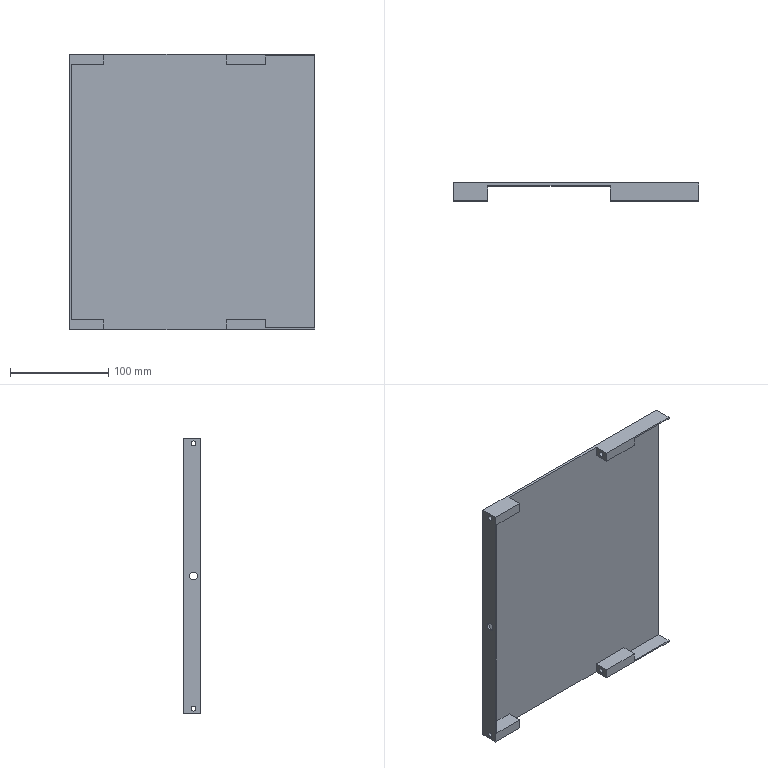Component | SolidWorks | SlideTablePlatform-1 | 1 solid | 32 faces | box 250 x 18 x 280 mm | volume 239541 mm3 | plane 22 | cylinder 10 | commonest cylinder face diameters 5 x8 8 x2
build123d program:
from build123d import *

# Parameters (mm, degrees)
SKETCH1_W           = 250
SKETCH1_H           = 280
BOSS_EXTRUDE1_DEPTH = 1.5
SKETCH2_W           = 35
SKETCH2_H           = 10
SKETCH2_W_2         = 40
BOSS_EXTRUDE2_DEPTH = 15
SKETCH3_R           = 2.5
CUT_EXTRUDE1_DEPTH  = 245.688
SKETCH4_W           = 50
SKETCH4_H           = 1.5
SKETCH4_W_2         = 2
SKETCH4_H_2         = 260
SKETCH4_H_3         = 1.549
BOSS_EXTRUDE3_DEPTH = 15
SKETCH5_R           = 4
CUT_EXTRUDE2_DEPTH  = 10


with BuildPart() as part:
    # Sketch1 → Boss-Extrude1 (new, symmetric)
    with BuildSketch(Plane(origin=(0, 0, 0), x_dir=(1, 0, 0), z_dir=(0, 1, 0))):
        Rectangle(SKETCH1_W, SKETCH1_H)
    extrude(amount=BOSS_EXTRUDE1_DEPTH, both=True)

    # Sketch2 → Boss-Extrude2 (add)
    with BuildSketch(Plane.XZ.offset(1.5)):
        with Locations((107.5, 135)):
            Rectangle(SKETCH2_W, SKETCH2_H)
        with Locations((107.5, -135)):
            Rectangle(SKETCH2_W, SKETCH2_H)
        with Locations((-55, 135)):
            Rectangle(SKETCH2_W_2, SKETCH2_H)
        with Locations((-55, -135)):
            Rectangle(SKETCH2_W_2, SKETCH2_H)
    extrude(amount=BOSS_EXTRUDE2_DEPTH)

    # Sketch3 → Cut-Extrude1 (cut, through all)
    with BuildSketch(Plane.ZY.offset(75)):
        with Locations((-135, -9)):
            Circle(SKETCH3_R)
        with Locations((135, -9)):
            Circle(SKETCH3_R)
    extrude(amount=-CUT_EXTRUDE1_DEPTH, mode=Mode.SUBTRACT)

    # Sketch4 → Boss-Extrude3 (add)
    with BuildSketch(Plane.XZ.offset(1.5)):
        with Locations((-100, -139.25)):
            Rectangle(SKETCH4_W, SKETCH4_H)
        with Locations((124, 0)):
            Rectangle(SKETCH4_W_2, SKETCH4_H_2)
        with Locations((-100, 139.225)):
            Rectangle(SKETCH4_W, SKETCH4_H_3)
    extrude(amount=BOSS_EXTRUDE3_DEPTH)

    # Sketch5 → Cut-Extrude2 (cut)
    with BuildSketch(Plane(origin=(125, 0, 0), x_dir=(0, 0, -1), z_dir=(1, 0, 0))):
        with Locations((0, -9)):
            Circle(SKETCH5_R)
    extrude(amount=-CUT_EXTRUDE2_DEPTH, mode=Mode.SUBTRACT)


solid = part.part

# Placed as in the assembly
solid = solid.moved(Location((157.663, 229, -10), (-180, 0, 180)))
STEP:
#1=COLOUR_RGB('',0.7922,0.8196,0.9333);
#2=FILL_AREA_STYLE_COLOUR('',#1);
#3=FILL_AREA_STYLE('',(#2));
#4=SURFACE_STYLE_FILL_AREA(#3);
#5=SURFACE_SIDE_STYLE('',(#4));
#6=SURFACE_STYLE_USAGE(.BOTH.,#5);
#7=PRESENTATION_STYLE_ASSIGNMENT((#6));
#8=CARTESIAN_POINT('',(1.365,8.661,-0.5512));
#9=VERTEX_POINT('',#8);
#10=CARTESIAN_POINT('',(1.365,8.661,-0.2362));
#11=VERTEX_POINT('',#10);
#12=CARTESIAN_POINT('',(1.365,8.661,-0.3937));
#13=DIRECTION('',(-1.,-0.,-0.));
#14=DIRECTION('',(-0.,0.,1.));
#15=AXIS2_PLACEMENT_3D('',#12,#13,#14);
#16=CIRCLE('',#15,0.1575);
#17=EDGE_CURVE('',#9,#11,#16,.T.);
#18=ORIENTED_EDGE('',*,*,#17,.F.);
#19=CARTESIAN_POINT('',(1.286,8.661,-0.5512));
#20=VERTEX_POINT('',#19);
#21=CARTESIAN_POINT('',(1.68,8.661,-0.5512));
#22=DIRECTION('',(-1.,-0.,-0.));
#23=VECTOR('',#22,39.37);
#24=LINE('',#21,#23);
#25=EDGE_CURVE('',#9,#20,#24,.T.);
#26=ORIENTED_EDGE('',*,*,#25,.T.);
#27=CARTESIAN_POINT('',(1.286,8.661,-0.2362));
#28=VERTEX_POINT('',#27);
#29=CARTESIAN_POINT('',(1.286,8.661,-0.3937));
#30=DIRECTION('',(-1.,-0.,-0.));
#31=DIRECTION('',(-0.,0.,1.));
#32=AXIS2_PLACEMENT_3D('',#29,#30,#31);
#33=CIRCLE('',#32,0.1575);
#34=EDGE_CURVE('',#20,#28,#33,.T.);
#35=ORIENTED_EDGE('',*,*,#34,.T.);
#36=CARTESIAN_POINT('',(1.68,8.661,-0.2362));
#37=DIRECTION('',(-1.,-0.,-0.));
#38=VECTOR('',#37,39.37);
#39=LINE('',#36,#38);
#40=EDGE_CURVE('',#11,#28,#39,.T.);
#41=ORIENTED_EDGE('',*,*,#40,.F.);
#42=EDGE_LOOP('',(#18,#26,#35,#41));
#43=FACE_OUTER_BOUND('',#42,.T.);
#44=CARTESIAN_POINT('',(1.68,8.661,-0.3937));
#45=DIRECTION('',(-1.,-0.,-0.));
#46=DIRECTION('',(-0.,0.,1.));
#47=AXIS2_PLACEMENT_3D('',#44,#45,#46);
#48=CYLINDRICAL_SURFACE('',#47,0.1575);
#49=ADVANCED_FACE('',(#43),#48,.F.);
#50=CARTESIAN_POINT('',(1.286,8.661,-5.61));
#51=VERTEX_POINT('',#50);
#52=CARTESIAN_POINT('',(1.286,8.661,-5.807));
#53=VERTEX_POINT('',#52);
#54=CARTESIAN_POINT('',(1.286,8.661,-5.709));
#55=DIRECTION('',(1.,0.,-0.));
#56=DIRECTION('',(0.,0.,-1.));
#57=AXIS2_PLACEMENT_3D('',#54,#55,#56);
#58=CIRCLE('',#57,0.09843);
#59=EDGE_CURVE('',#51,#53,#58,.T.);
#60=ORIENTED_EDGE('',*,*,#59,.F.);
#61=CARTESIAN_POINT('',(2.664,8.661,-5.61));
#62=VERTEX_POINT('',#61);
#63=CARTESIAN_POINT('',(1.286,8.661,-5.61));
#64=DIRECTION('',(1.,0.,-0.));
#65=VECTOR('',#64,39.37);
#66=LINE('',#63,#65);
#67=EDGE_CURVE('',#51,#62,#66,.T.);
#68=ORIENTED_EDGE('',*,*,#67,.T.);
#69=CARTESIAN_POINT('',(2.664,8.661,-5.807));
#70=VERTEX_POINT('',#69);
#71=CARTESIAN_POINT('',(2.664,8.661,-5.709));
#72=DIRECTION('',(-1.,-0.,-0.));
#73=DIRECTION('',(0.,0.,1.));
#74=AXIS2_PLACEMENT_3D('',#71,#72,#73);
#75=CIRCLE('',#74,0.09843);
#76=EDGE_CURVE('',#70,#62,#75,.T.);
#77=ORIENTED_EDGE('',*,*,#76,.F.);
#78=CARTESIAN_POINT('',(1.286,8.661,-5.807));
#79=DIRECTION('',(1.,0.,-0.));
#80=VECTOR('',#79,39.37);
#81=LINE('',#78,#80);
#82=EDGE_CURVE('',#53,#70,#81,.T.);
#83=ORIENTED_EDGE('',*,*,#82,.F.);
#84=EDGE_LOOP('',(#60,#68,#77,#83));
#85=FACE_OUTER_BOUND('',#84,.T.);
#86=CARTESIAN_POINT('',(1.286,8.661,-5.709));
#87=DIRECTION('',(1.,0.,-0.));
#88=DIRECTION('',(0.,0.,-1.));
#89=AXIS2_PLACEMENT_3D('',#86,#87,#88);
#90=CYLINDRICAL_SURFACE('',#89,0.09843);
#91=ADVANCED_FACE('',(#85),#90,.F.);
#92=CARTESIAN_POINT('',(1.286,8.661,5.02));
#93=VERTEX_POINT('',#92);
#94=CARTESIAN_POINT('',(1.286,8.661,4.823));
#95=VERTEX_POINT('',#94);
#96=CARTESIAN_POINT('',(1.286,8.661,4.921));
#97=DIRECTION('',(1.,0.,-0.));
#98=DIRECTION('',(0.,0.,-1.));
#99=AXIS2_PLACEMENT_3D('',#96,#97,#98);
#100=CIRCLE('',#99,0.09843);
#101=EDGE_CURVE('',#93,#95,#100,.T.);
#102=ORIENTED_EDGE('',*,*,#101,.F.);
#103=CARTESIAN_POINT('',(2.664,8.661,5.02));
#104=VERTEX_POINT('',#103);
#105=CARTESIAN_POINT('',(1.286,8.661,5.02));
#106=DIRECTION('',(1.,0.,-0.));
#107=VECTOR('',#106,39.37);
#108=LINE('',#105,#107);
#109=EDGE_CURVE('',#93,#104,#108,.T.);
#110=ORIENTED_EDGE('',*,*,#109,.T.);
#111=CARTESIAN_POINT('',(2.664,8.661,4.823));
#112=VERTEX_POINT('',#111);
#113=CARTESIAN_POINT('',(2.664,8.661,4.921));
#114=DIRECTION('',(-1.,-0.,0.));
#115=DIRECTION('',(0.,0.,1.));
#116=AXIS2_PLACEMENT_3D('',#113,#114,#115);
#117=CIRCLE('',#116,0.09843);
#118=EDGE_CURVE('',#112,#104,#117,.T.);
#119=ORIENTED_EDGE('',*,*,#118,.F.);
#120=CARTESIAN_POINT('',(1.286,8.661,4.823));
#121=DIRECTION('',(1.,0.,-0.));
#122=VECTOR('',#121,39.37);
#123=LINE('',#120,#122);
#124=EDGE_CURVE('',#95,#112,#123,.T.);
#125=ORIENTED_EDGE('',*,*,#124,.F.);
#126=EDGE_LOOP('',(#102,#110,#119,#125));
#127=FACE_OUTER_BOUND('',#126,.T.);
#128=CARTESIAN_POINT('',(1.286,8.661,4.921));
#129=DIRECTION('',(1.,0.,-0.));
#130=DIRECTION('',(0.,0.,-1.));
#131=AXIS2_PLACEMENT_3D('',#128,#129,#130);
#132=CYLINDRICAL_SURFACE('',#131,0.09843);
#133=ADVANCED_FACE('',(#127),#132,.F.);
#134=CARTESIAN_POINT('',(7.585,8.661,-5.61));
#135=VERTEX_POINT('',#134);
#136=CARTESIAN_POINT('',(7.585,8.661,-5.807));
#137=VERTEX_POINT('',#136);
#138=CARTESIAN_POINT('',(7.585,8.661,-5.709));
#139=DIRECTION('',(1.,0.,0.));
#140=DIRECTION('',(0.,0.,-1.));
#141=AXIS2_PLACEMENT_3D('',#138,#139,#140);
#142=CIRCLE('',#141,0.09843);
#143=EDGE_CURVE('',#135,#137,#142,.T.);
#144=ORIENTED_EDGE('',*,*,#143,.F.);
#145=CARTESIAN_POINT('',(9.16,8.661,-5.61));
#146=VERTEX_POINT('',#145);
#147=CARTESIAN_POINT('',(1.286,8.661,-5.61));
#148=DIRECTION('',(1.,0.,-0.));
#149=VECTOR('',#148,39.37);
#150=LINE('',#147,#149);
#151=EDGE_CURVE('',#135,#146,#150,.T.);
#152=ORIENTED_EDGE('',*,*,#151,.T.);
#153=CARTESIAN_POINT('',(9.16,8.661,-5.807));
#154=VERTEX_POINT('',#153);
#155=CARTESIAN_POINT('',(9.16,8.661,-5.709));
#156=DIRECTION('',(1.,0.,-0.));
#157=DIRECTION('',(0.,0.,-1.));
#158=AXIS2_PLACEMENT_3D('',#155,#156,#157);
#159=CIRCLE('',#158,0.09843);
#160=EDGE_CURVE('',#146,#154,#159,.T.);
#161=ORIENTED_EDGE('',*,*,#160,.T.);
#162=CARTESIAN_POINT('',(1.286,8.661,-5.807));
#163=DIRECTION('',(1.,0.,-0.));
#164=VECTOR('',#163,39.37);
#165=LINE('',#162,#164);
#166=EDGE_CURVE('',#137,#154,#165,.T.);
#167=ORIENTED_EDGE('',*,*,#166,.F.);
#168=EDGE_LOOP('',(#144,#152,#161,#167));
#169=FACE_OUTER_BOUND('',#168,.T.);
#170=CARTESIAN_POINT('',(1.286,8.661,-5.709));
#171=DIRECTION('',(1.,0.,-0.));
#172=DIRECTION('',(0.,0.,-1.));
#173=AXIS2_PLACEMENT_3D('',#170,#171,#172);
#174=CYLINDRICAL_SURFACE('',#173,0.09843);
#175=ADVANCED_FACE('',(#169),#174,.F.);
#176=CARTESIAN_POINT('',(7.585,8.661,5.02));
#177=VERTEX_POINT('',#176);
#178=CARTESIAN_POINT('',(7.585,8.661,4.823));
#179=VERTEX_POINT('',#178);
#180=CARTESIAN_POINT('',(7.585,8.661,4.921));
#181=DIRECTION('',(1.,0.,0.));
#182=DIRECTION('',(0.,0.,-1.));
#183=AXIS2_PLACEMENT_3D('',#180,#181,#182);
#184=CIRCLE('',#183,0.09843);
#185=EDGE_CURVE('',#177,#179,#184,.T.);
#186=ORIENTED_EDGE('',*,*,#185,.F.);
#187=CARTESIAN_POINT('',(9.16,8.661,5.02));
#188=VERTEX_POINT('',#187);
#189=CARTESIAN_POINT('',(1.286,8.661,5.02));
#190=DIRECTION('',(1.,0.,-0.));
#191=VECTOR('',#190,39.37);
#192=LINE('',#189,#191);
#193=EDGE_CURVE('',#177,#188,#192,.T.);
#194=ORIENTED_EDGE('',*,*,#193,.T.);
#195=CARTESIAN_POINT('',(9.16,8.661,4.823));
#196=VERTEX_POINT('',#195);
#197=CARTESIAN_POINT('',(9.16,8.661,4.921));
#198=DIRECTION('',(1.,0.,-0.));
#199=DIRECTION('',(0.,0.,-1.));
#200=AXIS2_PLACEMENT_3D('',#197,#198,#199);
#201=CIRCLE('',#200,0.09843);
#202=EDGE_CURVE('',#188,#196,#201,.T.);
#203=ORIENTED_EDGE('',*,*,#202,.T.);
#204=CARTESIAN_POINT('',(1.286,8.661,4.823));
#205=DIRECTION('',(1.,0.,-0.));
#206=VECTOR('',#205,39.37);
#207=LINE('',#204,#206);
#208=EDGE_CURVE('',#179,#196,#207,.T.);
#209=ORIENTED_EDGE('',*,*,#208,.F.);
#210=EDGE_LOOP('',(#186,#194,#203,#209));
#211=FACE_OUTER_BOUND('',#210,.T.);
#212=CARTESIAN_POINT('',(1.286,8.661,4.921));
#213=DIRECTION('',(1.,0.,-0.));
#214=DIRECTION('',(0.,0.,-1.));
#215=AXIS2_PLACEMENT_3D('',#212,#213,#214);
#216=CYLINDRICAL_SURFACE('',#215,0.09843);
#217=ADVANCED_FACE('',(#211),#216,.F.);
#218=CARTESIAN_POINT('',(11.128,8.957,-5.845));
#219=VERTEX_POINT('',#218);
#220=CARTESIAN_POINT('',(9.16,8.957,-5.845));
#221=VERTEX_POINT('',#220);
#222=CARTESIAN_POINT('',(9.16,8.957,-5.845));
#223=DIRECTION('',(-1.,-0.,-0.));
#224=VECTOR('',#223,39.37);
#225=LINE('',#222,#224);
#226=EDGE_CURVE('',#219,#221,#225,.T.);
#227=ORIENTED_EDGE('',*,*,#226,.F.);
#228=CARTESIAN_POINT('',(11.128,8.957,5.059));
#229=VERTEX_POINT('',#228);
#230=CARTESIAN_POINT('',(11.128,8.957,5.118));
#231=DIRECTION('',(0.,-0.,-1.));
#232=VECTOR('',#231,39.37);
#233=LINE('',#230,#232);
#234=EDGE_CURVE('',#229,#219,#233,.T.);
#235=ORIENTED_EDGE('',*,*,#234,.F.);
#236=CARTESIAN_POINT('',(9.16,8.957,5.059));
#237=VERTEX_POINT('',#236);
#238=CARTESIAN_POINT('',(9.16,8.957,5.059));
#239=DIRECTION('',(1.,0.,0.));
#240=VECTOR('',#239,39.37);
#241=LINE('',#238,#240);
#242=EDGE_CURVE('',#237,#229,#241,.T.);
#243=ORIENTED_EDGE('',*,*,#242,.F.);
#244=CARTESIAN_POINT('',(9.16,8.957,4.724));
#245=VERTEX_POINT('',#244);
#246=CARTESIAN_POINT('',(9.16,8.957,5.118));
#247=DIRECTION('',(-0.,0.,1.));
#248=VECTOR('',#247,39.37);
#249=LINE('',#246,#248);
#250=EDGE_CURVE('',#245,#237,#249,.T.);
#251=ORIENTED_EDGE('',*,*,#250,.F.);
#252=CARTESIAN_POINT('',(7.585,8.957,4.724));
#253=VERTEX_POINT('',#252);
#254=CARTESIAN_POINT('',(7.585,8.957,4.724));
#255=DIRECTION('',(1.,0.,0.));
#256=VECTOR('',#255,39.37);
#257=LINE('',#254,#256);
#258=EDGE_CURVE('',#253,#245,#257,.T.);
#259=ORIENTED_EDGE('',*,*,#258,.F.);
#260=CARTESIAN_POINT('',(7.585,8.957,5.118));
#261=VERTEX_POINT('',#260);
#262=CARTESIAN_POINT('',(7.585,8.957,5.118));
#263=DIRECTION('',(0.,-0.,-1.));
#264=VECTOR('',#263,39.37);
#265=LINE('',#262,#264);
#266=EDGE_CURVE('',#261,#253,#265,.T.);
#267=ORIENTED_EDGE('',*,*,#266,.F.);
#268=CARTESIAN_POINT('',(2.664,8.957,5.118));
#269=VERTEX_POINT('',#268);
#270=CARTESIAN_POINT('',(11.128,8.957,5.118));
#271=DIRECTION('',(1.,0.,0.));
#272=VECTOR('',#271,39.37);
#273=LINE('',#270,#272);
#274=EDGE_CURVE('',#269,#261,#273,.T.);
#275=ORIENTED_EDGE('',*,*,#274,.F.);
#276=CARTESIAN_POINT('',(2.664,8.957,4.724));
#277=VERTEX_POINT('',#276);
#278=CARTESIAN_POINT('',(2.664,8.957,5.118));
#279=DIRECTION('',(0.,0.,1.));
#280=VECTOR('',#279,39.37);
#281=LINE('',#278,#280);
#282=EDGE_CURVE('',#277,#269,#281,.T.);
#283=ORIENTED_EDGE('',*,*,#282,.F.);
#284=CARTESIAN_POINT('',(1.365,8.957,4.724));
#285=VERTEX_POINT('',#284);
#286=CARTESIAN_POINT('',(1.286,8.957,4.724));
#287=DIRECTION('',(1.,0.,0.));
#288=VECTOR('',#287,39.37);
#289=LINE('',#286,#288);
#290=EDGE_CURVE('',#285,#277,#289,.T.);
#291=ORIENTED_EDGE('',*,*,#290,.F.);
#292=CARTESIAN_POINT('',(1.365,8.957,-5.512));
#293=VERTEX_POINT('',#292);
#294=CARTESIAN_POINT('',(1.365,8.957,4.724));
#295=DIRECTION('',(-0.,0.,1.));
#296=VECTOR('',#295,39.37);
#297=LINE('',#294,#296);
#298=EDGE_CURVE('',#293,#285,#297,.T.);
#299=ORIENTED_EDGE('',*,*,#298,.F.);
#300=CARTESIAN_POINT('',(2.664,8.957,-5.512));
#301=VERTEX_POINT('',#300);
#302=CARTESIAN_POINT('',(1.286,8.957,-5.512));
#303=DIRECTION('',(-1.,-0.,-0.));
#304=VECTOR('',#303,39.37);
#305=LINE('',#302,#304);
#306=EDGE_CURVE('',#301,#293,#305,.T.);
#307=ORIENTED_EDGE('',*,*,#306,.F.);
#308=CARTESIAN_POINT('',(2.664,8.957,-5.906));
#309=VERTEX_POINT('',#308);
#310=CARTESIAN_POINT('',(2.664,8.957,-5.906));
#311=DIRECTION('',(-0.,0.,1.));
#312=VECTOR('',#311,39.37);
#313=LINE('',#310,#312);
#314=EDGE_CURVE('',#309,#301,#313,.T.);
#315=ORIENTED_EDGE('',*,*,#314,.F.);
#316=CARTESIAN_POINT('',(7.585,8.957,-5.906));
#317=VERTEX_POINT('',#316);
#318=CARTESIAN_POINT('',(11.128,8.957,-5.906));
#319=DIRECTION('',(-1.,-0.,-0.));
#320=VECTOR('',#319,39.37);
#321=LINE('',#318,#320);
#322=EDGE_CURVE('',#317,#309,#321,.T.);
#323=ORIENTED_EDGE('',*,*,#322,.F.);
#324=CARTESIAN_POINT('',(7.585,8.957,-5.512));
#325=VERTEX_POINT('',#324);
#326=CARTESIAN_POINT('',(7.585,8.957,-5.906));
#327=DIRECTION('',(0.,-0.,-1.));
#328=VECTOR('',#327,39.37);
#329=LINE('',#326,#328);
#330=EDGE_CURVE('',#325,#317,#329,.T.);
#331=ORIENTED_EDGE('',*,*,#330,.F.);
#332=CARTESIAN_POINT('',(9.16,8.957,-5.512));
#333=VERTEX_POINT('',#332);
#334=CARTESIAN_POINT('',(9.16,8.957,-5.512));
#335=DIRECTION('',(-1.,-0.,-0.));
#336=VECTOR('',#335,39.37);
#337=LINE('',#334,#336);
#338=EDGE_CURVE('',#333,#325,#337,.T.);
#339=ORIENTED_EDGE('',*,*,#338,.F.);
#340=CARTESIAN_POINT('',(9.16,8.957,-5.906));
#341=DIRECTION('',(-0.,0.,1.));
#342=VECTOR('',#341,39.37);
#343=LINE('',#340,#342);
#344=EDGE_CURVE('',#221,#333,#343,.T.);
#345=ORIENTED_EDGE('',*,*,#344,.F.);
#346=EDGE_LOOP('',(#227,#235,#243,#251,#259,#267,#275,#283,#291,#299,#307,#315,#323,#331,#339,#345));
#347=FACE_OUTER_BOUND('',#346,.T.);
#348=CARTESIAN_POINT('',(6.207,8.957,-0.3937));
#349=DIRECTION('',(-0.,1.,-0.));
#350=DIRECTION('',(0.,-0.,-1.));
#351=AXIS2_PLACEMENT_3D('',#348,#349,#350);
#352=PLANE('',#351);
#353=ADVANCED_FACE('',(#347),#352,.F.);
#354=CARTESIAN_POINT('',(9.16,8.661,-5.709));
#355=DIRECTION('',(1.,0.,-0.));
#356=DIRECTION('',(0.,0.,-1.));
#357=AXIS2_PLACEMENT_3D('',#354,#355,#356);
#358=CIRCLE('',#357,0.09843);
#359=EDGE_CURVE('',#154,#146,#358,.T.);
#360=ORIENTED_EDGE('',*,*,#359,.F.);
#361=ORIENTED_EDGE('',*,*,#160,.F.);
#362=EDGE_LOOP('',(#360,#361));
#363=FACE_BOUND('',#362,.T.);
#364=CARTESIAN_POINT('',(9.16,8.366,-5.845));
#365=VERTEX_POINT('',#364);
#366=CARTESIAN_POINT('',(9.16,-1.87,-5.845));
#367=DIRECTION('',(-0.,1.,-0.));
#368=VECTOR('',#367,39.37);
#369=LINE('',#366,#368);
#370=EDGE_CURVE('',#365,#221,#369,.T.);
#371=ORIENTED_EDGE('',*,*,#370,.T.);
#372=ORIENTED_EDGE('',*,*,#344,.T.);
#373=CARTESIAN_POINT('',(9.16,8.366,-5.512));
#374=VERTEX_POINT('',#373);
#375=CARTESIAN_POINT('',(9.16,8.366,-5.512));
#376=DIRECTION('',(-0.,1.,-0.));
#377=VECTOR('',#376,39.37);
#378=LINE('',#375,#377);
#379=EDGE_CURVE('',#374,#333,#378,.T.);
#380=ORIENTED_EDGE('',*,*,#379,.F.);
#381=CARTESIAN_POINT('',(9.16,8.366,-5.906));
#382=DIRECTION('',(-0.,0.,1.));
#383=VECTOR('',#382,39.37);
#384=LINE('',#381,#383);
#385=EDGE_CURVE('',#365,#374,#384,.T.);
#386=ORIENTED_EDGE('',*,*,#385,.F.);
#387=EDGE_LOOP('',(#371,#372,#380,#386));
#388=FACE_OUTER_BOUND('',#387,.T.);
#389=CARTESIAN_POINT('',(9.16,8.366,-5.906));
#390=DIRECTION('',(-1.,-0.,-0.));
#391=DIRECTION('',(-0.,0.,1.));
#392=AXIS2_PLACEMENT_3D('',#389,#390,#391);
#393=PLANE('',#392);
#394=ADVANCED_FACE('',(#363,#388),#393,.F.);
#395=CARTESIAN_POINT('',(1.365,8.366,-5.512));
#396=VERTEX_POINT('',#395);
#397=CARTESIAN_POINT('',(1.365,-1.87,-5.512));
#398=DIRECTION('',(-0.,1.,-0.));
#399=VECTOR('',#398,39.37);
#400=LINE('',#397,#399);
#401=EDGE_CURVE('',#396,#293,#400,.T.);
#402=ORIENTED_EDGE('',*,*,#401,.F.);
#403=CARTESIAN_POINT('',(2.664,8.366,-5.512));
#404=VERTEX_POINT('',#403);
#405=CARTESIAN_POINT('',(1.286,8.366,-5.512));
#406=DIRECTION('',(-1.,-0.,-0.));
#407=VECTOR('',#406,39.37);
#408=LINE('',#405,#407);
#409=EDGE_CURVE('',#404,#396,#408,.T.);
#410=ORIENTED_EDGE('',*,*,#409,.F.);
#411=CARTESIAN_POINT('',(2.664,8.366,-5.512));
#412=DIRECTION('',(-0.,1.,-0.));
#413=VECTOR('',#412,39.37);
#414=LINE('',#411,#413);
#415=EDGE_CURVE('',#404,#301,#414,.T.);
#416=ORIENTED_EDGE('',*,*,#415,.T.);
#417=ORIENTED_EDGE('',*,*,#306,.T.);
#418=EDGE_LOOP('',(#402,#410,#416,#417));
#419=FACE_OUTER_BOUND('',#418,.T.);
#420=CARTESIAN_POINT('',(1.286,8.366,-5.512));
#421=DIRECTION('',(0.,-0.,-1.));
#422=DIRECTION('',(-1.,-0.,-0.));
#423=AXIS2_PLACEMENT_3D('',#420,#421,#422);
#424=PLANE('',#423);
#425=ADVANCED_FACE('',(#419),#424,.F.);
#426=CARTESIAN_POINT('',(1.365,8.366,4.724));
#427=VERTEX_POINT('',#426);
#428=CARTESIAN_POINT('',(1.365,-1.87,4.724));
#429=DIRECTION('',(-0.,1.,-0.));
#430=VECTOR('',#429,39.37);
#431=LINE('',#428,#430);
#432=EDGE_CURVE('',#427,#285,#431,.T.);
#433=ORIENTED_EDGE('',*,*,#432,.T.);
#434=ORIENTED_EDGE('',*,*,#290,.T.);
#435=CARTESIAN_POINT('',(2.664,8.366,4.724));
#436=VERTEX_POINT('',#435);
#437=CARTESIAN_POINT('',(2.664,8.366,4.724));
#438=DIRECTION('',(-0.,1.,-0.));
#439=VECTOR('',#438,39.37);
#440=LINE('',#437,#439);
#441=EDGE_CURVE('',#436,#277,#440,.T.);
#442=ORIENTED_EDGE('',*,*,#441,.F.);
#443=CARTESIAN_POINT('',(1.286,8.366,4.724));
#444=DIRECTION('',(1.,0.,0.));
#445=VECTOR('',#444,39.37);
#446=LINE('',#443,#445);
#447=EDGE_CURVE('',#427,#436,#446,.T.);
#448=ORIENTED_EDGE('',*,*,#447,.F.);
#449=EDGE_LOOP('',(#433,#434,#442,#448));
#450=FACE_OUTER_BOUND('',#449,.T.);
#451=CARTESIAN_POINT('',(1.286,8.366,4.724));
#452=DIRECTION('',(-0.,0.,1.));
#453=DIRECTION('',(1.,0.,0.));
#454=AXIS2_PLACEMENT_3D('',#451,#452,#453);
#455=PLANE('',#454);
#456=ADVANCED_FACE('',(#450),#455,.F.);
#457=CARTESIAN_POINT('',(9.16,8.661,4.921));
#458=DIRECTION('',(1.,0.,-0.));
#459=DIRECTION('',(0.,0.,-1.));
#460=AXIS2_PLACEMENT_3D('',#457,#458,#459);
#461=CIRCLE('',#460,0.09843);
#462=EDGE_CURVE('',#196,#188,#461,.T.);
#463=ORIENTED_EDGE('',*,*,#462,.F.);
#464=ORIENTED_EDGE('',*,*,#202,.F.);
#465=EDGE_LOOP('',(#463,#464));
#466=FACE_BOUND('',#465,.T.);
#467=CARTESIAN_POINT('',(9.16,8.366,5.059));
#468=VERTEX_POINT('',#467);
#469=CARTESIAN_POINT('',(9.16,-1.87,5.059));
#470=DIRECTION('',(-0.,1.,-0.));
#471=VECTOR('',#470,39.37);
#472=LINE('',#469,#471);
#473=EDGE_CURVE('',#468,#237,#472,.T.);
#474=ORIENTED_EDGE('',*,*,#473,.F.);
#475=CARTESIAN_POINT('',(9.16,8.366,4.724));
#476=VERTEX_POINT('',#475);
#477=CARTESIAN_POINT('',(9.16,8.366,5.118));
#478=DIRECTION('',(-0.,0.,1.));
#479=VECTOR('',#478,39.37);
#480=LINE('',#477,#479);
#481=EDGE_CURVE('',#476,#468,#480,.T.);
#482=ORIENTED_EDGE('',*,*,#481,.F.);
#483=CARTESIAN_POINT('',(9.16,8.366,4.724));
#484=DIRECTION('',(-0.,1.,-0.));
#485=VECTOR('',#484,39.37);
#486=LINE('',#483,#485);
#487=EDGE_CURVE('',#476,#245,#486,.T.);
#488=ORIENTED_EDGE('',*,*,#487,.T.);
#489=ORIENTED_EDGE('',*,*,#250,.T.);
#490=EDGE_LOOP('',(#474,#482,#488,#489));
#491=FACE_OUTER_BOUND('',#490,.T.);
#492=CARTESIAN_POINT('',(9.16,8.366,5.118));
#493=DIRECTION('',(-1.,-0.,-0.));
#494=DIRECTION('',(-0.,0.,1.));
#495=AXIS2_PLACEMENT_3D('',#492,#493,#494);
#496=PLANE('',#495);
#497=ADVANCED_FACE('',(#466,#491),#496,.F.);
#498=CARTESIAN_POINT('',(1.286,8.661,-0.3937));
#499=DIRECTION('',(-1.,-0.,-0.));
#500=DIRECTION('',(-0.,0.,1.));
#501=AXIS2_PLACEMENT_3D('',#498,#499,#500);
#502=CIRCLE('',#501,0.1575);
#503=EDGE_CURVE('',#28,#20,#502,.T.);
#504=ORIENTED_EDGE('',*,*,#503,.F.);
#505=ORIENTED_EDGE('',*,*,#34,.F.);
#506=EDGE_LOOP('',(#504,#505));
#507=FACE_BOUND('',#506,.T.);
#508=CARTESIAN_POINT('',(1.286,8.661,4.921));
#509=DIRECTION('',(1.,0.,-0.));
#510=DIRECTION('',(0.,0.,-1.));
#511=AXIS2_PLACEMENT_3D('',#508,#509,#510);
#512=CIRCLE('',#511,0.09843);
#513=EDGE_CURVE('',#95,#93,#512,.T.);
#514=ORIENTED_EDGE('',*,*,#513,.T.);
#515=ORIENTED_EDGE('',*,*,#101,.T.);
#516=EDGE_LOOP('',(#514,#515));
#517=FACE_BOUND('',#516,.T.);
#518=CARTESIAN_POINT('',(1.286,8.661,-5.709));
#519=DIRECTION('',(1.,0.,-0.));
#520=DIRECTION('',(0.,0.,-1.));
#521=AXIS2_PLACEMENT_3D('',#518,#519,#520);
#522=CIRCLE('',#521,0.09843);
#523=EDGE_CURVE('',#53,#51,#522,.T.);
#524=ORIENTED_EDGE('',*,*,#523,.T.);
#525=ORIENTED_EDGE('',*,*,#59,.T.);
#526=EDGE_LOOP('',(#524,#525));
#527=FACE_BOUND('',#526,.T.);
#528=CARTESIAN_POINT('',(1.286,9.075,-5.906));
#529=VERTEX_POINT('',#528);
#530=CARTESIAN_POINT('',(1.286,8.366,-5.906));
#531=VERTEX_POINT('',#530);
#532=CARTESIAN_POINT('',(1.286,9.075,-5.906));
#533=DIRECTION('',(0.,-1.,0.));
#534=VECTOR('',#533,39.37);
#535=LINE('',#532,#534);
#536=EDGE_CURVE('',#529,#531,#535,.T.);
#537=ORIENTED_EDGE('',*,*,#536,.T.);
#538=CARTESIAN_POINT('',(1.286,8.366,5.118));
#539=VERTEX_POINT('',#538);
#540=CARTESIAN_POINT('',(1.286,8.366,-5.906));
#541=DIRECTION('',(0.,-0.,-1.));
#542=VECTOR('',#541,39.37);
#543=LINE('',#540,#542);
#544=EDGE_CURVE('',#539,#531,#543,.T.);
#545=ORIENTED_EDGE('',*,*,#544,.F.);
#546=CARTESIAN_POINT('',(1.286,9.075,5.118));
#547=VERTEX_POINT('',#546);
#548=CARTESIAN_POINT('',(1.286,9.075,5.118));
#549=DIRECTION('',(0.,-1.,0.));
#550=VECTOR('',#549,39.37);
#551=LINE('',#548,#550);
#552=EDGE_CURVE('',#547,#539,#551,.T.);
#553=ORIENTED_EDGE('',*,*,#552,.F.);
#554=CARTESIAN_POINT('',(1.286,9.075,5.118));
#555=DIRECTION('',(-0.,0.,1.));
#556=VECTOR('',#555,39.37);
#557=LINE('',#554,#556);
#558=EDGE_CURVE('',#529,#547,#557,.T.);
#559=ORIENTED_EDGE('',*,*,#558,.F.);
#560=EDGE_LOOP('',(#537,#545,#553,#559));
#561=FACE_OUTER_BOUND('',#560,.T.);
#562=CARTESIAN_POINT('',(1.286,9.075,5.118));
#563=DIRECTION('',(1.,0.,0.));
#564=DIRECTION('',(0.,-0.,-1.));
#565=AXIS2_PLACEMENT_3D('',#562,#563,#564);
#566=PLANE('',#565);
#567=ADVANCED_FACE('',(#507,#517,#527,#561),#566,.F.);
#568=CARTESIAN_POINT('',(11.128,8.366,5.118));
#569=VERTEX_POINT('',#568);
#570=CARTESIAN_POINT('',(7.585,8.366,5.118));
#571=VERTEX_POINT('',#570);
#572=CARTESIAN_POINT('',(7.585,8.366,5.118));
#573=DIRECTION('',(-1.,-0.,-0.));
#574=VECTOR('',#573,39.37);
#575=LINE('',#572,#574);
#576=EDGE_CURVE('',#569,#571,#575,.T.);
#577=ORIENTED_EDGE('',*,*,#576,.F.);
#578=CARTESIAN_POINT('',(11.128,9.075,5.118));
#579=VERTEX_POINT('',#578);
#580=CARTESIAN_POINT('',(11.128,9.075,5.118));
#581=DIRECTION('',(0.,-1.,0.));
#582=VECTOR('',#581,39.37);
#583=LINE('',#580,#582);
#584=EDGE_CURVE('',#579,#569,#583,.T.);
#585=ORIENTED_EDGE('',*,*,#584,.F.);
#586=CARTESIAN_POINT('',(11.128,9.075,5.118));
#587=DIRECTION('',(1.,0.,0.));
#588=VECTOR('',#587,39.37);
#589=LINE('',#586,#588);
#590=EDGE_CURVE('',#547,#579,#589,.T.);
#591=ORIENTED_EDGE('',*,*,#590,.F.);
#592=ORIENTED_EDGE('',*,*,#552,.T.);
#593=CARTESIAN_POINT('',(2.664,8.366,5.118));
#594=VERTEX_POINT('',#593);
#595=CARTESIAN_POINT('',(1.286,8.366,5.118));
#596=DIRECTION('',(-1.,-0.,-0.));
#597=VECTOR('',#596,39.37);
#598=LINE('',#595,#597);
#599=EDGE_CURVE('',#594,#539,#598,.T.);
#600=ORIENTED_EDGE('',*,*,#599,.F.);
#601=CARTESIAN_POINT('',(2.664,8.366,5.118));
#602=DIRECTION('',(-0.,1.,-0.));
#603=VECTOR('',#602,39.37);
#604=LINE('',#601,#603);
#605=EDGE_CURVE('',#594,#269,#604,.T.);
#606=ORIENTED_EDGE('',*,*,#605,.T.);
#607=ORIENTED_EDGE('',*,*,#274,.T.);
#608=CARTESIAN_POINT('',(7.585,8.366,5.118));
#609=DIRECTION('',(-0.,1.,-0.));
#610=VECTOR('',#609,39.37);
#611=LINE('',#608,#610);
#612=EDGE_CURVE('',#571,#261,#611,.T.);
#613=ORIENTED_EDGE('',*,*,#612,.F.);
#614=EDGE_LOOP('',(#577,#585,#591,#592,#600,#606,#607,#613));
#615=FACE_OUTER_BOUND('',#614,.T.);
#616=CARTESIAN_POINT('',(11.128,9.075,5.118));
#617=DIRECTION('',(0.,-0.,-1.));
#618=DIRECTION('',(-1.,-0.,-0.));
#619=AXIS2_PLACEMENT_3D('',#616,#617,#618);
#620=PLANE('',#619);
#621=ADVANCED_FACE('',(#615),#620,.F.);
#622=ORIENTED_EDGE('',*,*,#584,.T.);
#623=CARTESIAN_POINT('',(11.128,8.366,5.059));
#624=VERTEX_POINT('',#623);
#625=CARTESIAN_POINT('',(11.128,8.366,5.118));
#626=DIRECTION('',(0.,-0.,-1.));
#627=VECTOR('',#626,39.37);
#628=LINE('',#625,#627);
#629=EDGE_CURVE('',#569,#624,#628,.T.);
#630=ORIENTED_EDGE('',*,*,#629,.T.);
#631=CARTESIAN_POINT('',(11.128,-1.87,5.059));
#632=DIRECTION('',(-0.,1.,-0.));
#633=VECTOR('',#632,39.37);
#634=LINE('',#631,#633);
#635=EDGE_CURVE('',#624,#229,#634,.T.);
#636=ORIENTED_EDGE('',*,*,#635,.T.);
#637=ORIENTED_EDGE('',*,*,#234,.T.);
#638=CARTESIAN_POINT('',(11.128,8.366,-5.845));
#639=VERTEX_POINT('',#638);
#640=CARTESIAN_POINT('',(11.128,-1.87,-5.845));
#641=DIRECTION('',(-0.,1.,-0.));
#642=VECTOR('',#641,39.37);
#643=LINE('',#640,#642);
#644=EDGE_CURVE('',#639,#219,#643,.T.);
#645=ORIENTED_EDGE('',*,*,#644,.F.);
#646=CARTESIAN_POINT('',(11.128,8.366,-5.906));
#647=VERTEX_POINT('',#646);
#648=CARTESIAN_POINT('',(11.128,8.366,-5.845));
#649=DIRECTION('',(0.,-0.,-1.));
#650=VECTOR('',#649,39.37);
#651=LINE('',#648,#650);
#652=EDGE_CURVE('',#639,#647,#651,.T.);
#653=ORIENTED_EDGE('',*,*,#652,.T.);
#654=CARTESIAN_POINT('',(11.128,9.075,-5.906));
#655=VERTEX_POINT('',#654);
#656=CARTESIAN_POINT('',(11.128,9.075,-5.906));
#657=DIRECTION('',(0.,-1.,0.));
#658=VECTOR('',#657,39.37);
#659=LINE('',#656,#658);
#660=EDGE_CURVE('',#655,#647,#659,.T.);
#661=ORIENTED_EDGE('',*,*,#660,.F.);
#662=CARTESIAN_POINT('',(11.128,9.075,5.118));
#663=DIRECTION('',(0.,-0.,-1.));
#664=VECTOR('',#663,39.37);
#665=LINE('',#662,#664);
#666=EDGE_CURVE('',#579,#655,#665,.T.);
#667=ORIENTED_EDGE('',*,*,#666,.F.);
#668=EDGE_LOOP('',(#622,#630,#636,#637,#645,#653,#661,#667));
#669=FACE_OUTER_BOUND('',#668,.T.);
#670=CARTESIAN_POINT('',(11.128,9.075,5.118));
#671=DIRECTION('',(-1.,-0.,-0.));
#672=DIRECTION('',(-0.,0.,1.));
#673=AXIS2_PLACEMENT_3D('',#670,#671,#672);
#674=PLANE('',#673);
#675=ADVANCED_FACE('',(#669),#674,.F.);
#676=ORIENTED_EDGE('',*,*,#660,.T.);
#677=CARTESIAN_POINT('',(7.585,8.366,-5.906));
#678=VERTEX_POINT('',#677);
#679=CARTESIAN_POINT('',(9.16,8.366,-5.906));
#680=DIRECTION('',(1.,0.,0.));
#681=VECTOR('',#680,39.37);
#682=LINE('',#679,#681);
#683=EDGE_CURVE('',#678,#647,#682,.T.);
#684=ORIENTED_EDGE('',*,*,#683,.F.);
#685=CARTESIAN_POINT('',(7.585,8.366,-5.906));
#686=DIRECTION('',(-0.,1.,-0.));
#687=VECTOR('',#686,39.37);
#688=LINE('',#685,#687);
#689=EDGE_CURVE('',#678,#317,#688,.T.);
#690=ORIENTED_EDGE('',*,*,#689,.T.);
#691=ORIENTED_EDGE('',*,*,#322,.T.);
#692=CARTESIAN_POINT('',(2.664,8.366,-5.906));
#693=VERTEX_POINT('',#692);
#694=CARTESIAN_POINT('',(2.664,8.366,-5.906));
#695=DIRECTION('',(-0.,1.,-0.));
#696=VECTOR('',#695,39.37);
#697=LINE('',#694,#696);
#698=EDGE_CURVE('',#693,#309,#697,.T.);
#699=ORIENTED_EDGE('',*,*,#698,.F.);
#700=CARTESIAN_POINT('',(1.286,8.366,-5.906));
#701=DIRECTION('',(1.,0.,0.));
#702=VECTOR('',#701,39.37);
#703=LINE('',#700,#702);
#704=EDGE_CURVE('',#531,#693,#703,.T.);
#705=ORIENTED_EDGE('',*,*,#704,.F.);
#706=ORIENTED_EDGE('',*,*,#536,.F.);
#707=CARTESIAN_POINT('',(11.128,9.075,-5.906));
#708=DIRECTION('',(-1.,-0.,-0.));
#709=VECTOR('',#708,39.37);
#710=LINE('',#707,#709);
#711=EDGE_CURVE('',#655,#529,#710,.T.);
#712=ORIENTED_EDGE('',*,*,#711,.F.);
#713=EDGE_LOOP('',(#676,#684,#690,#691,#699,#705,#706,#712));
#714=FACE_OUTER_BOUND('',#713,.T.);
#715=CARTESIAN_POINT('',(11.128,9.075,-5.906));
#716=DIRECTION('',(-0.,0.,1.));
#717=DIRECTION('',(1.,0.,0.));
#718=AXIS2_PLACEMENT_3D('',#715,#716,#717);
#719=PLANE('',#718);
#720=ADVANCED_FACE('',(#714),#719,.F.);
#721=ORIENTED_EDGE('',*,*,#558,.T.);
#722=ORIENTED_EDGE('',*,*,#590,.T.);
#723=ORIENTED_EDGE('',*,*,#666,.T.);
#724=ORIENTED_EDGE('',*,*,#711,.T.);
#725=EDGE_LOOP('',(#721,#722,#723,#724));
#726=FACE_OUTER_BOUND('',#725,.T.);
#727=CARTESIAN_POINT('',(6.207,9.075,-0.3937));
#728=DIRECTION('',(-0.,1.,-0.));
#729=DIRECTION('',(0.,-0.,-1.));
#730=AXIS2_PLACEMENT_3D('',#727,#728,#729);
#731=PLANE('',#730);
#732=ADVANCED_FACE('',(#726),#731,.T.);
#733=ORIENTED_EDGE('',*,*,#76,.T.);
#734=CARTESIAN_POINT('',(2.664,8.661,-5.709));
#735=DIRECTION('',(-1.,-0.,-0.));
#736=DIRECTION('',(0.,0.,1.));
#737=AXIS2_PLACEMENT_3D('',#734,#735,#736);
#738=CIRCLE('',#737,0.09843);
#739=EDGE_CURVE('',#62,#70,#738,.T.);
#740=ORIENTED_EDGE('',*,*,#739,.T.);
#741=EDGE_LOOP('',(#733,#740));
#742=FACE_BOUND('',#741,.T.);
#743=ORIENTED_EDGE('',*,*,#314,.T.);
#744=ORIENTED_EDGE('',*,*,#415,.F.);
#745=CARTESIAN_POINT('',(2.664,8.366,-5.906));
#746=DIRECTION('',(-0.,0.,1.));
#747=VECTOR('',#746,39.37);
#748=LINE('',#745,#747);
#749=EDGE_CURVE('',#693,#404,#748,.T.);
#750=ORIENTED_EDGE('',*,*,#749,.F.);
#751=ORIENTED_EDGE('',*,*,#698,.T.);
#752=EDGE_LOOP('',(#743,#744,#750,#751));
#753=FACE_OUTER_BOUND('',#752,.T.);
#754=CARTESIAN_POINT('',(2.664,8.366,-5.906));
#755=DIRECTION('',(-1.,-0.,-0.));
#756=DIRECTION('',(-0.,0.,1.));
#757=AXIS2_PLACEMENT_3D('',#754,#755,#756);
#758=PLANE('',#757);
#759=ADVANCED_FACE('',(#742,#753),#758,.F.);
#760=ORIENTED_EDGE('',*,*,#544,.T.);
#761=ORIENTED_EDGE('',*,*,#704,.T.);
#762=ORIENTED_EDGE('',*,*,#749,.T.);
#763=ORIENTED_EDGE('',*,*,#409,.T.);
#764=CARTESIAN_POINT('',(1.365,8.366,4.724));
#765=DIRECTION('',(0.,-0.,-1.));
#766=VECTOR('',#765,39.37);
#767=LINE('',#764,#766);
#768=EDGE_CURVE('',#427,#396,#767,.T.);
#769=ORIENTED_EDGE('',*,*,#768,.F.);
#770=ORIENTED_EDGE('',*,*,#447,.T.);
#771=CARTESIAN_POINT('',(2.664,8.366,5.118));
#772=DIRECTION('',(0.,0.,1.));
#773=VECTOR('',#772,39.37);
#774=LINE('',#771,#773);
#775=EDGE_CURVE('',#436,#594,#774,.T.);
#776=ORIENTED_EDGE('',*,*,#775,.T.);
#777=ORIENTED_EDGE('',*,*,#599,.T.);
#778=EDGE_LOOP('',(#760,#761,#762,#763,#769,#770,#776,#777));
#779=FACE_OUTER_BOUND('',#778,.T.);
#780=CARTESIAN_POINT('',(6.207,8.366,-0.3937));
#781=DIRECTION('',(-0.,1.,-0.));
#782=DIRECTION('',(0.,-0.,-1.));
#783=AXIS2_PLACEMENT_3D('',#780,#781,#782);
#784=PLANE('',#783);
#785=ADVANCED_FACE('',(#779),#784,.F.);
#786=ORIENTED_EDGE('',*,*,#118,.T.);
#787=CARTESIAN_POINT('',(2.664,8.661,4.921));
#788=DIRECTION('',(-1.,-0.,0.));
#789=DIRECTION('',(0.,0.,1.));
#790=AXIS2_PLACEMENT_3D('',#787,#788,#789);
#791=CIRCLE('',#790,0.09843);
#792=EDGE_CURVE('',#104,#112,#791,.T.);
#793=ORIENTED_EDGE('',*,*,#792,.T.);
#794=EDGE_LOOP('',(#786,#793));
#795=FACE_BOUND('',#794,.T.);
#796=ORIENTED_EDGE('',*,*,#282,.T.);
#797=ORIENTED_EDGE('',*,*,#605,.F.);
#798=ORIENTED_EDGE('',*,*,#775,.F.);
#799=ORIENTED_EDGE('',*,*,#441,.T.);
#800=EDGE_LOOP('',(#796,#797,#798,#799));
#801=FACE_OUTER_BOUND('',#800,.T.);
#802=CARTESIAN_POINT('',(2.664,8.366,5.118));
#803=DIRECTION('',(-1.,-0.,0.));
#804=DIRECTION('',(0.,0.,1.));
#805=AXIS2_PLACEMENT_3D('',#802,#803,#804);
#806=PLANE('',#805);
#807=ADVANCED_FACE('',(#795,#801),#806,.F.);
#808=CARTESIAN_POINT('',(7.585,8.661,-5.709));
#809=DIRECTION('',(1.,0.,0.));
#810=DIRECTION('',(0.,0.,-1.));
#811=AXIS2_PLACEMENT_3D('',#808,#809,#810);
#812=CIRCLE('',#811,0.09843);
#813=EDGE_CURVE('',#137,#135,#812,.T.);
#814=ORIENTED_EDGE('',*,*,#813,.T.);
#815=ORIENTED_EDGE('',*,*,#143,.T.);
#816=EDGE_LOOP('',(#814,#815));
#817=FACE_BOUND('',#816,.T.);
#818=ORIENTED_EDGE('',*,*,#330,.T.);
#819=ORIENTED_EDGE('',*,*,#689,.F.);
#820=CARTESIAN_POINT('',(7.585,8.366,-5.512));
#821=VERTEX_POINT('',#820);
#822=CARTESIAN_POINT('',(7.585,8.366,-5.906));
#823=DIRECTION('',(0.,-0.,-1.));
#824=VECTOR('',#823,39.37);
#825=LINE('',#822,#824);
#826=EDGE_CURVE('',#821,#678,#825,.T.);
#827=ORIENTED_EDGE('',*,*,#826,.F.);
#828=CARTESIAN_POINT('',(7.585,8.366,-5.512));
#829=DIRECTION('',(-0.,1.,-0.));
#830=VECTOR('',#829,39.37);
#831=LINE('',#828,#830);
#832=EDGE_CURVE('',#821,#325,#831,.T.);
#833=ORIENTED_EDGE('',*,*,#832,.T.);
#834=EDGE_LOOP('',(#818,#819,#827,#833));
#835=FACE_OUTER_BOUND('',#834,.T.);
#836=CARTESIAN_POINT('',(7.585,8.366,-5.906));
#837=DIRECTION('',(1.,0.,0.));
#838=DIRECTION('',(0.,-0.,-1.));
#839=AXIS2_PLACEMENT_3D('',#836,#837,#838);
#840=PLANE('',#839);
#841=ADVANCED_FACE('',(#817,#835),#840,.F.);
#842=ORIENTED_EDGE('',*,*,#338,.T.);
#843=ORIENTED_EDGE('',*,*,#832,.F.);
#844=CARTESIAN_POINT('',(9.16,8.366,-5.512));
#845=DIRECTION('',(-1.,-0.,-0.));
#846=VECTOR('',#845,39.37);
#847=LINE('',#844,#846);
#848=EDGE_CURVE('',#374,#821,#847,.T.);
#849=ORIENTED_EDGE('',*,*,#848,.F.);
#850=ORIENTED_EDGE('',*,*,#379,.T.);
#851=EDGE_LOOP('',(#842,#843,#849,#850));
#852=FACE_OUTER_BOUND('',#851,.T.);
#853=CARTESIAN_POINT('',(9.16,8.366,-5.512));
#854=DIRECTION('',(0.,-0.,-1.));
#855=DIRECTION('',(-1.,-0.,-0.));
#856=AXIS2_PLACEMENT_3D('',#853,#854,#855);
#857=PLANE('',#856);
#858=ADVANCED_FACE('',(#852),#857,.F.);
#859=ORIENTED_EDGE('',*,*,#826,.T.);
#860=ORIENTED_EDGE('',*,*,#683,.T.);
#861=ORIENTED_EDGE('',*,*,#652,.F.);
#862=CARTESIAN_POINT('',(9.16,8.366,-5.845));
#863=DIRECTION('',(1.,0.,0.));
#864=VECTOR('',#863,39.37);
#865=LINE('',#862,#864);
#866=EDGE_CURVE('',#365,#639,#865,.T.);
#867=ORIENTED_EDGE('',*,*,#866,.F.);
#868=ORIENTED_EDGE('',*,*,#385,.T.);
#869=ORIENTED_EDGE('',*,*,#848,.T.);
#870=EDGE_LOOP('',(#859,#860,#861,#867,#868,#869));
#871=FACE_OUTER_BOUND('',#870,.T.);
#872=CARTESIAN_POINT('',(6.207,8.366,-0.3937));
#873=DIRECTION('',(0.,-1.,0.));
#874=DIRECTION('',(-0.,0.,1.));
#875=AXIS2_PLACEMENT_3D('',#872,#873,#874);
#876=PLANE('',#875);
#877=ADVANCED_FACE('',(#871),#876,.T.);
#878=CARTESIAN_POINT('',(7.585,8.661,4.921));
#879=DIRECTION('',(1.,0.,0.));
#880=DIRECTION('',(0.,0.,-1.));
#881=AXIS2_PLACEMENT_3D('',#878,#879,#880);
#882=CIRCLE('',#881,0.09843);
#883=EDGE_CURVE('',#179,#177,#882,.T.);
#884=ORIENTED_EDGE('',*,*,#883,.T.);
#885=ORIENTED_EDGE('',*,*,#185,.T.);
#886=EDGE_LOOP('',(#884,#885));
#887=FACE_BOUND('',#886,.T.);
#888=ORIENTED_EDGE('',*,*,#266,.T.);
#889=CARTESIAN_POINT('',(7.585,8.366,4.724));
#890=VERTEX_POINT('',#889);
#891=CARTESIAN_POINT('',(7.585,8.366,4.724));
#892=DIRECTION('',(-0.,1.,-0.));
#893=VECTOR('',#892,39.37);
#894=LINE('',#891,#893);
#895=EDGE_CURVE('',#890,#253,#894,.T.);
#896=ORIENTED_EDGE('',*,*,#895,.F.);
#897=CARTESIAN_POINT('',(7.585,8.366,5.118));
#898=DIRECTION('',(0.,-0.,-1.));
#899=VECTOR('',#898,39.37);
#900=LINE('',#897,#899);
#901=EDGE_CURVE('',#571,#890,#900,.T.);
#902=ORIENTED_EDGE('',*,*,#901,.F.);
#903=ORIENTED_EDGE('',*,*,#612,.T.);
#904=EDGE_LOOP('',(#888,#896,#902,#903));
#905=FACE_OUTER_BOUND('',#904,.T.);
#906=CARTESIAN_POINT('',(7.585,8.366,5.118));
#907=DIRECTION('',(1.,0.,0.));
#908=DIRECTION('',(0.,-0.,-1.));
#909=AXIS2_PLACEMENT_3D('',#906,#907,#908);
#910=PLANE('',#909);
#911=ADVANCED_FACE('',(#887,#905),#910,.F.);
#912=ORIENTED_EDGE('',*,*,#258,.T.);
#913=ORIENTED_EDGE('',*,*,#487,.F.);
#914=CARTESIAN_POINT('',(7.585,8.366,4.724));
#915=DIRECTION('',(1.,0.,0.));
#916=VECTOR('',#915,39.37);
#917=LINE('',#914,#916);
#918=EDGE_CURVE('',#890,#476,#917,.T.);
#919=ORIENTED_EDGE('',*,*,#918,.F.);
#920=ORIENTED_EDGE('',*,*,#895,.T.);
#921=EDGE_LOOP('',(#912,#913,#919,#920));
#922=FACE_OUTER_BOUND('',#921,.T.);
#923=CARTESIAN_POINT('',(7.585,8.366,4.724));
#924=DIRECTION('',(-0.,0.,1.));
#925=DIRECTION('',(1.,0.,0.));
#926=AXIS2_PLACEMENT_3D('',#923,#924,#925);
#927=PLANE('',#926);
#928=ADVANCED_FACE('',(#922),#927,.F.);
#929=ORIENTED_EDGE('',*,*,#481,.T.);
#930=CARTESIAN_POINT('',(9.16,8.366,5.059));
#931=DIRECTION('',(-1.,-0.,-0.));
#932=VECTOR('',#931,39.37);
#933=LINE('',#930,#932);
#934=EDGE_CURVE('',#624,#468,#933,.T.);
#935=ORIENTED_EDGE('',*,*,#934,.F.);
#936=ORIENTED_EDGE('',*,*,#629,.F.);
#937=ORIENTED_EDGE('',*,*,#576,.T.);
#938=ORIENTED_EDGE('',*,*,#901,.T.);
#939=ORIENTED_EDGE('',*,*,#918,.T.);
#940=EDGE_LOOP('',(#929,#935,#936,#937,#938,#939));
#941=FACE_OUTER_BOUND('',#940,.T.);
#942=CARTESIAN_POINT('',(6.207,8.366,-0.3937));
#943=DIRECTION('',(0.,-1.,0.));
#944=DIRECTION('',(-0.,0.,1.));
#945=AXIS2_PLACEMENT_3D('',#942,#943,#944);
#946=PLANE('',#945);
#947=ADVANCED_FACE('',(#941),#946,.T.);
#948=ORIENTED_EDGE('',*,*,#193,.F.);
#949=ORIENTED_EDGE('',*,*,#883,.F.);
#950=ORIENTED_EDGE('',*,*,#208,.T.);
#951=ORIENTED_EDGE('',*,*,#462,.T.);
#952=EDGE_LOOP('',(#948,#949,#950,#951));
#953=FACE_OUTER_BOUND('',#952,.T.);
#954=CARTESIAN_POINT('',(1.286,8.661,4.921));
#955=DIRECTION('',(1.,0.,-0.));
#956=DIRECTION('',(0.,0.,-1.));
#957=AXIS2_PLACEMENT_3D('',#954,#955,#956);
#958=CYLINDRICAL_SURFACE('',#957,0.09843);
#959=ADVANCED_FACE('',(#953),#958,.F.);
#960=ORIENTED_EDGE('',*,*,#151,.F.);
#961=ORIENTED_EDGE('',*,*,#813,.F.);
#962=ORIENTED_EDGE('',*,*,#166,.T.);
#963=ORIENTED_EDGE('',*,*,#359,.T.);
#964=EDGE_LOOP('',(#960,#961,#962,#963));
#965=FACE_OUTER_BOUND('',#964,.T.);
#966=CARTESIAN_POINT('',(1.286,8.661,-5.709));
#967=DIRECTION('',(1.,0.,-0.));
#968=DIRECTION('',(0.,0.,-1.));
#969=AXIS2_PLACEMENT_3D('',#966,#967,#968);
#970=CYLINDRICAL_SURFACE('',#969,0.09843);
#971=ADVANCED_FACE('',(#965),#970,.F.);
#972=ORIENTED_EDGE('',*,*,#109,.F.);
#973=ORIENTED_EDGE('',*,*,#513,.F.);
#974=ORIENTED_EDGE('',*,*,#124,.T.);
#975=ORIENTED_EDGE('',*,*,#792,.F.);
#976=EDGE_LOOP('',(#972,#973,#974,#975));
#977=FACE_OUTER_BOUND('',#976,.T.);
#978=CARTESIAN_POINT('',(1.286,8.661,4.921));
#979=DIRECTION('',(1.,0.,-0.));
#980=DIRECTION('',(0.,0.,-1.));
#981=AXIS2_PLACEMENT_3D('',#978,#979,#980);
#982=CYLINDRICAL_SURFACE('',#981,0.09843);
#983=ADVANCED_FACE('',(#977),#982,.F.);
#984=ORIENTED_EDGE('',*,*,#67,.F.);
#985=ORIENTED_EDGE('',*,*,#523,.F.);
#986=ORIENTED_EDGE('',*,*,#82,.T.);
#987=ORIENTED_EDGE('',*,*,#739,.F.);
#988=EDGE_LOOP('',(#984,#985,#986,#987));
#989=FACE_OUTER_BOUND('',#988,.T.);
#990=CARTESIAN_POINT('',(1.286,8.661,-5.709));
#991=DIRECTION('',(1.,0.,-0.));
#992=DIRECTION('',(0.,0.,-1.));
#993=AXIS2_PLACEMENT_3D('',#990,#991,#992);
#994=CYLINDRICAL_SURFACE('',#993,0.09843);
#995=ADVANCED_FACE('',(#989),#994,.F.);
#996=ORIENTED_EDGE('',*,*,#635,.F.);
#997=ORIENTED_EDGE('',*,*,#934,.T.);
#998=ORIENTED_EDGE('',*,*,#473,.T.);
#999=ORIENTED_EDGE('',*,*,#242,.T.);
#1000=EDGE_LOOP('',(#996,#997,#998,#999));
#1001=FACE_OUTER_BOUND('',#1000,.T.);
#1002=CARTESIAN_POINT('',(9.16,-1.87,5.059));
#1003=DIRECTION('',(-0.,0.,1.));
#1004=DIRECTION('',(1.,0.,0.));
#1005=AXIS2_PLACEMENT_3D('',#1002,#1003,#1004);
#1006=PLANE('',#1005);
#1007=ADVANCED_FACE('',(#1001),#1006,.F.);
#1008=CARTESIAN_POINT('',(1.365,8.661,-0.3937));
#1009=DIRECTION('',(-1.,-0.,-0.));
#1010=DIRECTION('',(-0.,0.,1.));
#1011=AXIS2_PLACEMENT_3D('',#1008,#1009,#1010);
#1012=CIRCLE('',#1011,0.1575);
#1013=EDGE_CURVE('',#11,#9,#1012,.T.);
#1014=ORIENTED_EDGE('',*,*,#1013,.T.);
#1015=ORIENTED_EDGE('',*,*,#17,.T.);
#1016=EDGE_LOOP('',(#1014,#1015));
#1017=FACE_BOUND('',#1016,.T.);
#1018=ORIENTED_EDGE('',*,*,#432,.F.);
#1019=ORIENTED_EDGE('',*,*,#768,.T.);
#1020=ORIENTED_EDGE('',*,*,#401,.T.);
#1021=ORIENTED_EDGE('',*,*,#298,.T.);
#1022=EDGE_LOOP('',(#1018,#1019,#1020,#1021));
#1023=FACE_OUTER_BOUND('',#1022,.T.);
#1024=CARTESIAN_POINT('',(1.365,-1.87,4.724));
#1025=DIRECTION('',(-1.,-0.,-0.));
#1026=DIRECTION('',(-0.,0.,1.));
#1027=AXIS2_PLACEMENT_3D('',#1024,#1025,#1026);
#1028=PLANE('',#1027);
#1029=ADVANCED_FACE('',(#1017,#1023),#1028,.F.);
#1030=ORIENTED_EDGE('',*,*,#370,.F.);
#1031=ORIENTED_EDGE('',*,*,#866,.T.);
#1032=ORIENTED_EDGE('',*,*,#644,.T.);
#1033=ORIENTED_EDGE('',*,*,#226,.T.);
#1034=EDGE_LOOP('',(#1030,#1031,#1032,#1033));
#1035=FACE_OUTER_BOUND('',#1034,.T.);
#1036=CARTESIAN_POINT('',(9.16,-1.87,-5.845));
#1037=DIRECTION('',(0.,-0.,-1.));
#1038=DIRECTION('',(-1.,-0.,-0.));
#1039=AXIS2_PLACEMENT_3D('',#1036,#1037,#1038);
#1040=PLANE('',#1039);
#1041=ADVANCED_FACE('',(#1035),#1040,.F.);
#1042=ORIENTED_EDGE('',*,*,#25,.F.);
#1043=ORIENTED_EDGE('',*,*,#1013,.F.);
#1044=ORIENTED_EDGE('',*,*,#40,.T.);
#1045=ORIENTED_EDGE('',*,*,#503,.T.);
#1046=EDGE_LOOP('',(#1042,#1043,#1044,#1045));
#1047=FACE_OUTER_BOUND('',#1046,.T.);
#1048=CARTESIAN_POINT('',(1.68,8.661,-0.3937));
#1049=DIRECTION('',(-1.,-0.,-0.));
#1050=DIRECTION('',(-0.,0.,1.));
#1051=AXIS2_PLACEMENT_3D('',#1048,#1049,#1050);
#1052=CYLINDRICAL_SURFACE('',#1051,0.1575);
#1053=ADVANCED_FACE('',(#1047),#1052,.F.);
#1054=CLOSED_SHELL('',(#49,#91,#133,#175,#217,#353,#394,#425,#456,#497,#567,#621,#675,#720,#732,#759,#785,#807,#841,#858,#877,#911,#928,#947,#959,#971,#983,#995,#1007,#1029,#1041,#1053));
#1055=MANIFOLD_SOLID_BREP('',#1054);
#1056=STYLED_ITEM('',(#7),#1055);
#1057=PRESENTATION_LAYER_ASSIGNMENT('','',(#1056));
#1058=CARTESIAN_POINT('',(0.,0.,0.));
#1059=DIRECTION('',(0.,0.,1.));
#1060=DIRECTION('',(1.,0.,0.));
#1061=AXIS2_PLACEMENT_3D('',#1058,#1059,#1060);
#1062=(LENGTH_UNIT()NAMED_UNIT(*)SI_UNIT($,.METRE.));
#1063=LENGTH_MEASURE_WITH_UNIT(LENGTH_MEASURE(0.0254),#1062);
#1064=DIMENSIONAL_EXPONENTS(1.,0.,0.,0.,0.,0.,0.);
#1065=(CONVERSION_BASED_UNIT('',#1063)LENGTH_UNIT()NAMED_UNIT(#1064));
#1066=UNCERTAINTY_MEASURE_WITH_UNIT(LENGTH_MEASURE(0.00001),#1065,'','');
#1067=(NAMED_UNIT(*)PLANE_ANGLE_UNIT()SI_UNIT($,.RADIAN.));
#1068=(NAMED_UNIT(*)SI_UNIT($,.STERADIAN.)SOLID_ANGLE_UNIT());
#1069=(GEOMETRIC_REPRESENTATION_CONTEXT(3)GLOBAL_UNCERTAINTY_ASSIGNED_CONTEXT((#1066))GLOBAL_UNIT_ASSIGNED_CONTEXT((#1065,#1067,#1068))REPRESENTATION_CONTEXT('',''));
#1070=ADVANCED_BREP_SHAPE_REPRESENTATION('',(#1055,#1061),#1069);
#1071=(LENGTH_UNIT()NAMED_UNIT(*)SI_UNIT($,.METRE.));
#1072=LENGTH_MEASURE_WITH_UNIT(LENGTH_MEASURE(0.0254),#1071);
#1073=DIMENSIONAL_EXPONENTS(1.,0.,0.,0.,0.,0.,0.);
#1074=(CONVERSION_BASED_UNIT('',#1072)LENGTH_UNIT()NAMED_UNIT(#1073));
#1075=UNCERTAINTY_MEASURE_WITH_UNIT(LENGTH_MEASURE(0.00001),#1074,'','');
#1076=(NAMED_UNIT(*)PLANE_ANGLE_UNIT()SI_UNIT($,.RADIAN.));
#1077=(NAMED_UNIT(*)SI_UNIT($,.STERADIAN.)SOLID_ANGLE_UNIT());
#1078=(GEOMETRIC_REPRESENTATION_CONTEXT(3)GLOBAL_UNCERTAINTY_ASSIGNED_CONTEXT((#1075))GLOBAL_UNIT_ASSIGNED_CONTEXT((#1074,#1076,#1077))REPRESENTATION_CONTEXT('',''));
#1079=MECHANICAL_DESIGN_GEOMETRIC_PRESENTATION_REPRESENTATION('',(#1056),#1078);